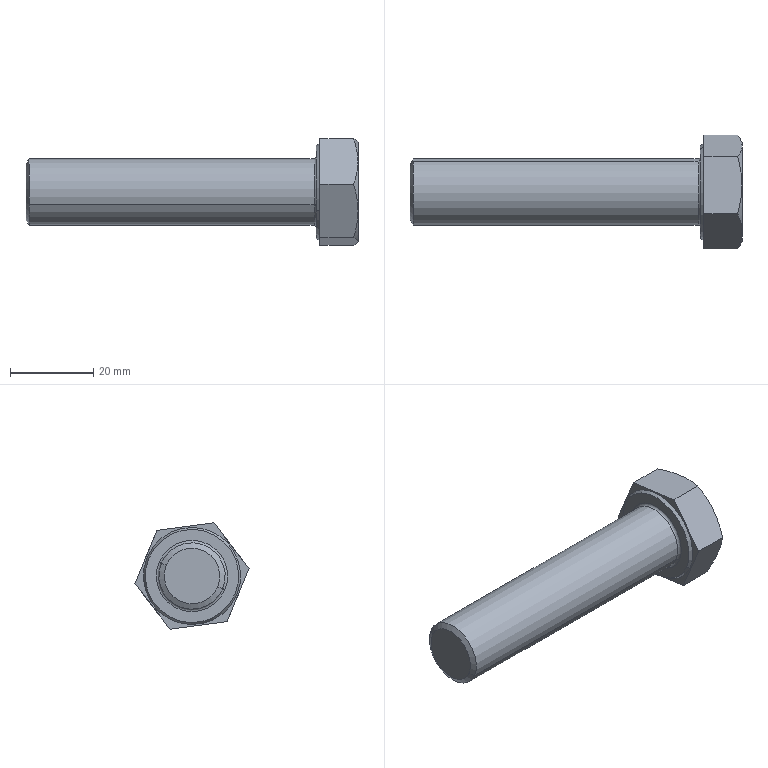Component | SolidWorks | GB_T5786-2000[HexHeadBoltFineThreadFullThreadM16_1.5_70]-1 | 1 solid | 24 faces | box 80 x 27.47 x 25.61 mm | volume 18960 mm3 | cone 10 | plane 10 | torus 2 | cylinder 2 | commonest cylinder face diameters 16 x2
STEP:
#1=COLOUR_RGB('',0.7922,0.8196,0.9333);
#2=FILL_AREA_STYLE_COLOUR('',#1);
#3=FILL_AREA_STYLE('',(#2));
#4=SURFACE_STYLE_FILL_AREA(#3);
#5=SURFACE_SIDE_STYLE('',(#4));
#6=SURFACE_STYLE_USAGE(.BOTH.,#5);
#7=PRESENTATION_STYLE_ASSIGNMENT((#6));
#8=CARTESIAN_POINT('',(-10.098,279.523,4.075));
#9=VERTEX_POINT('',#8);
#10=CARTESIAN_POINT('',(-10.098,280.01,4.277));
#11=VERTEX_POINT('',#10);
#12=CARTESIAN_POINT('',(-10.098,279.766,4.176));
#13=DIRECTION('',(1.,0.,0.));
#14=DIRECTION('',(0.,-0.9242,-0.3818));
#15=AXIS2_PLACEMENT_3D('',#12,#13,#14);
#16=CIRCLE('',#15,0.2638);
#17=EDGE_CURVE('',#9,#11,#16,.T.);
#18=ORIENTED_EDGE('',*,*,#17,.T.);
#19=CARTESIAN_POINT('',(-10.069,280.057,4.296));
#20=VERTEX_POINT('',#19);
#21=CARTESIAN_POINT('',(-10.069,280.057,4.296));
#22=DIRECTION('',(0.5,0.8004,0.3307));
#23=VECTOR('',#22,39.37);
#24=LINE('',#21,#23);
#25=EDGE_CURVE('',#11,#20,#24,.T.);
#26=ORIENTED_EDGE('',*,*,#25,.T.);
#27=CARTESIAN_POINT('',(-10.069,279.475,4.056));
#28=VERTEX_POINT('',#27);
#29=CARTESIAN_POINT('',(-10.069,279.766,4.176));
#30=DIRECTION('',(1.,0.,0.));
#31=DIRECTION('',(0.,-0.9242,-0.3818));
#32=AXIS2_PLACEMENT_3D('',#29,#30,#31);
#33=CIRCLE('',#32,0.315);
#34=EDGE_CURVE('',#28,#20,#33,.T.);
#35=ORIENTED_EDGE('',*,*,#34,.F.);
#36=CARTESIAN_POINT('',(-10.069,279.475,4.056));
#37=DIRECTION('',(0.5,-0.8004,-0.3307));
#38=VECTOR('',#37,39.37);
#39=LINE('',#36,#38);
#40=EDGE_CURVE('',#9,#28,#39,.T.);
#41=ORIENTED_EDGE('',*,*,#40,.F.);
#42=EDGE_LOOP('',(#18,#26,#35,#41));
#43=FACE_OUTER_BOUND('',#42,.T.);
#44=CARTESIAN_POINT('',(-10.069,279.766,4.176));
#45=DIRECTION('',(1.,0.,0.));
#46=DIRECTION('',(0.,-0.9242,-0.3818));
#47=AXIS2_PLACEMENT_3D('',#44,#45,#46);
#48=CONICAL_SURFACE('',#47,0.315,1.047);
#49=ADVANCED_FACE('',(#43),#48,.T.);
#50=CARTESIAN_POINT('',(-7.366,279.475,4.056));
#51=VERTEX_POINT('',#50);
#52=CARTESIAN_POINT('',(-7.366,280.057,4.296));
#53=VERTEX_POINT('',#52);
#54=CARTESIAN_POINT('',(-7.366,279.766,4.176));
#55=DIRECTION('',(-1.,0.,0.));
#56=DIRECTION('',(0.,0.9242,0.3818));
#57=AXIS2_PLACEMENT_3D('',#54,#55,#56);
#58=CIRCLE('',#57,0.315);
#59=EDGE_CURVE('',#51,#53,#58,.T.);
#60=ORIENTED_EDGE('',*,*,#59,.F.);
#61=CARTESIAN_POINT('',(-7.343,279.453,4.047));
#62=VERTEX_POINT('',#61);
#63=CARTESIAN_POINT('',(-7.366,279.453,4.047));
#64=DIRECTION('',(0.,0.3818,-0.9242));
#65=DIRECTION('',(0.,0.9242,0.3818));
#66=AXIS2_PLACEMENT_3D('',#63,#64,#65);
#67=CIRCLE('',#66,0.02362);
#68=EDGE_CURVE('',#51,#62,#67,.T.);
#69=ORIENTED_EDGE('',*,*,#68,.T.);
#70=CARTESIAN_POINT('',(-7.343,280.079,4.305));
#71=VERTEX_POINT('',#70);
#72=CARTESIAN_POINT('',(-7.343,279.766,4.176));
#73=DIRECTION('',(1.,0.,0.));
#74=DIRECTION('',(0.,0.9242,0.3818));
#75=AXIS2_PLACEMENT_3D('',#72,#73,#74);
#76=CIRCLE('',#75,0.3386);
#77=EDGE_CURVE('',#71,#62,#76,.T.);
#78=ORIENTED_EDGE('',*,*,#77,.F.);
#79=CARTESIAN_POINT('',(-7.366,280.079,4.305));
#80=DIRECTION('',(0.,-0.3818,0.9242));
#81=DIRECTION('',(0.,-0.9242,-0.3818));
#82=AXIS2_PLACEMENT_3D('',#79,#80,#81);
#83=CIRCLE('',#82,0.02362);
#84=EDGE_CURVE('',#53,#71,#83,.T.);
#85=ORIENTED_EDGE('',*,*,#84,.F.);
#86=EDGE_LOOP('',(#60,#69,#78,#85));
#87=FACE_OUTER_BOUND('',#86,.T.);
#88=CARTESIAN_POINT('',(-7.366,279.766,4.176));
#89=DIRECTION('',(-1.,0.,0.));
#90=DIRECTION('',(0.,0.9242,0.3818));
#91=AXIS2_PLACEMENT_3D('',#88,#89,#90);
#92=TOROIDAL_SURFACE('',#91,0.3386,0.02362);
#93=ADVANCED_FACE('',(#87),#92,.F.);
#94=CARTESIAN_POINT('',(-7.343,279.357,4.007));
#95=VERTEX_POINT('',#94);
#96=CARTESIAN_POINT('',(-7.343,280.176,4.345));
#97=VERTEX_POINT('',#96);
#98=CARTESIAN_POINT('',(-7.343,279.766,4.176));
#99=DIRECTION('',(1.,0.,0.));
#100=DIRECTION('',(0.,-0.9242,-0.3818));
#101=AXIS2_PLACEMENT_3D('',#98,#99,#100);
#102=CIRCLE('',#101,0.4427);
#103=EDGE_CURVE('',#95,#97,#102,.T.);
#104=ORIENTED_EDGE('',*,*,#103,.T.);
#105=CARTESIAN_POINT('',(-7.311,280.192,4.352));
#106=VERTEX_POINT('',#105);
#107=CARTESIAN_POINT('',(-7.311,280.192,4.352));
#108=DIRECTION('',(0.866,0.4621,0.1909));
#109=VECTOR('',#108,39.37);
#110=LINE('',#107,#109);
#111=EDGE_CURVE('',#97,#106,#110,.T.);
#112=ORIENTED_EDGE('',*,*,#111,.T.);
#113=CARTESIAN_POINT('',(-7.311,279.34,4.));
#114=VERTEX_POINT('',#113);
#115=CARTESIAN_POINT('',(-7.311,279.766,4.176));
#116=DIRECTION('',(1.,0.,0.));
#117=DIRECTION('',(0.,-0.9242,-0.3818));
#118=AXIS2_PLACEMENT_3D('',#115,#116,#117);
#119=CIRCLE('',#118,0.4609);
#120=EDGE_CURVE('',#114,#106,#119,.T.);
#121=ORIENTED_EDGE('',*,*,#120,.F.);
#122=CARTESIAN_POINT('',(-7.311,279.34,4.));
#123=DIRECTION('',(0.866,-0.4621,-0.1909));
#124=VECTOR('',#123,39.37);
#125=LINE('',#122,#124);
#126=EDGE_CURVE('',#95,#114,#125,.T.);
#127=ORIENTED_EDGE('',*,*,#126,.F.);
#128=EDGE_LOOP('',(#104,#112,#121,#127));
#129=FACE_OUTER_BOUND('',#128,.T.);
#130=CARTESIAN_POINT('',(-7.311,279.766,4.176));
#131=DIRECTION('',(1.,0.,0.));
#132=DIRECTION('',(0.,-0.9242,-0.3818));
#133=AXIS2_PLACEMENT_3D('',#130,#131,#132);
#134=CONICAL_SURFACE('',#133,0.4609,0.5236);
#135=ADVANCED_FACE('',(#129),#134,.T.);
#136=ORIENTED_EDGE('',*,*,#34,.T.);
#137=CARTESIAN_POINT('',(-6.949,280.057,4.296));
#138=DIRECTION('',(1.,0.,0.));
#139=VECTOR('',#138,39.37);
#140=LINE('',#137,#139);
#141=EDGE_CURVE('',#20,#53,#140,.T.);
#142=ORIENTED_EDGE('',*,*,#141,.T.);
#143=CARTESIAN_POINT('',(-7.366,279.766,4.176));
#144=DIRECTION('',(-1.,0.,0.));
#145=DIRECTION('',(0.,0.9242,0.3818));
#146=AXIS2_PLACEMENT_3D('',#143,#144,#145);
#147=CIRCLE('',#146,0.315);
#148=EDGE_CURVE('',#53,#51,#147,.T.);
#149=ORIENTED_EDGE('',*,*,#148,.T.);
#150=CARTESIAN_POINT('',(-6.949,279.475,4.056));
#151=DIRECTION('',(1.,0.,0.));
#152=VECTOR('',#151,39.37);
#153=LINE('',#150,#152);
#154=EDGE_CURVE('',#28,#51,#153,.T.);
#155=ORIENTED_EDGE('',*,*,#154,.F.);
#156=EDGE_LOOP('',(#136,#142,#149,#155));
#157=FACE_OUTER_BOUND('',#156,.T.);
#158=CARTESIAN_POINT('',(-6.949,279.766,4.176));
#159=DIRECTION('',(1.,0.,0.));
#160=DIRECTION('',(0.,-0.9242,-0.3818));
#161=AXIS2_PLACEMENT_3D('',#158,#159,#160);
#162=CYLINDRICAL_SURFACE('',#161,0.315);
#163=ADVANCED_FACE('',(#157),#162,.T.);
#164=ORIENTED_EDGE('',*,*,#141,.F.);
#165=CARTESIAN_POINT('',(-10.069,279.766,4.176));
#166=DIRECTION('',(1.,0.,0.));
#167=DIRECTION('',(0.,-0.9242,-0.3818));
#168=AXIS2_PLACEMENT_3D('',#165,#166,#167);
#169=CIRCLE('',#168,0.315);
#170=EDGE_CURVE('',#20,#28,#169,.T.);
#171=ORIENTED_EDGE('',*,*,#170,.T.);
#172=ORIENTED_EDGE('',*,*,#154,.T.);
#173=ORIENTED_EDGE('',*,*,#59,.T.);
#174=EDGE_LOOP('',(#164,#171,#172,#173));
#175=FACE_OUTER_BOUND('',#174,.T.);
#176=CARTESIAN_POINT('',(-6.949,279.766,4.176));
#177=DIRECTION('',(1.,0.,0.));
#178=DIRECTION('',(0.,-0.9242,-0.3818));
#179=AXIS2_PLACEMENT_3D('',#176,#177,#178);
#180=CYLINDRICAL_SURFACE('',#179,0.315);
#181=ADVANCED_FACE('',(#175),#180,.T.);
#182=CARTESIAN_POINT('',(-7.311,280.307,4.104));
#183=VERTEX_POINT('',#182);
#184=CARTESIAN_POINT('',(-7.311,279.975,3.672));
#185=VERTEX_POINT('',#184);
#186=CARTESIAN_POINT('',(-7.311,280.307,4.104));
#187=DIRECTION('',(0.,-0.6095,-0.7928));
#188=VECTOR('',#187,39.37);
#189=LINE('',#186,#188);
#190=EDGE_CURVE('',#183,#185,#189,.T.);
#191=ORIENTED_EDGE('',*,*,#190,.F.);
#192=CARTESIAN_POINT('',(-6.991,280.307,4.104));
#193=VERTEX_POINT('',#192);
#194=CARTESIAN_POINT('',(-7.343,280.307,4.104));
#195=DIRECTION('',(1.,0.,0.));
#196=VECTOR('',#195,39.37);
#197=LINE('',#194,#196);
#198=EDGE_CURVE('',#183,#193,#197,.T.);
#199=ORIENTED_EDGE('',*,*,#198,.T.);
#200=CARTESIAN_POINT('',(-6.949,280.141,3.888));
#201=VERTEX_POINT('',#200);
#202=CARTESIAN_POINT('',(-6.949,280.141,3.888));
#203=CARTESIAN_POINT('',(-6.949,280.155,3.906));
#204=CARTESIAN_POINT('',(-6.95,280.169,3.925));
#205=CARTESIAN_POINT('',(-6.954,280.197,3.961));
#206=CARTESIAN_POINT('',(-6.957,280.211,3.979));
#207=CARTESIAN_POINT('',(-6.968,280.253,4.033));
#208=CARTESIAN_POINT('',(-6.978,280.28,4.069));
#209=CARTESIAN_POINT('',(-6.991,280.307,4.104));
#210=B_SPLINE_CURVE_WITH_KNOTS('',3,(#202,#203,#204,#205,#206,#207,#208,#209),.UNSPECIFIED.,.F.,.F.,(4,2,2,4),(0.00701,0.008756,0.0105,0.01399),.UNSPECIFIED.);
#211=EDGE_CURVE('',#201,#193,#210,.T.);
#212=ORIENTED_EDGE('',*,*,#211,.F.);
#213=CARTESIAN_POINT('',(-6.991,279.975,3.672));
#214=VERTEX_POINT('',#213);
#215=CARTESIAN_POINT('',(-6.991,279.975,3.672));
#216=CARTESIAN_POINT('',(-6.978,280.002,3.707));
#217=CARTESIAN_POINT('',(-6.968,280.029,3.743));
#218=CARTESIAN_POINT('',(-6.953,280.085,3.815));
#219=CARTESIAN_POINT('',(-6.949,280.113,3.851));
#220=CARTESIAN_POINT('',(-6.949,280.141,3.888));
#221=B_SPLINE_CURVE_WITH_KNOTS('',3,(#215,#216,#217,#218,#219,#220),.UNSPECIFIED.,.F.,.F.,(4,2,4),(0.00000024,0.003505,0.00701),.UNSPECIFIED.);
#222=EDGE_CURVE('',#214,#201,#221,.T.);
#223=ORIENTED_EDGE('',*,*,#222,.F.);
#224=CARTESIAN_POINT('',(-7.343,279.975,3.672));
#225=DIRECTION('',(1.,0.,0.));
#226=VECTOR('',#225,39.37);
#227=LINE('',#224,#226);
#228=EDGE_CURVE('',#185,#214,#227,.T.);
#229=ORIENTED_EDGE('',*,*,#228,.F.);
#230=EDGE_LOOP('',(#191,#199,#212,#223,#229));
#231=FACE_OUTER_BOUND('',#230,.T.);
#232=CARTESIAN_POINT('',(-7.343,280.307,4.104));
#233=DIRECTION('',(0.,-0.7928,0.6095));
#234=DIRECTION('',(0.,0.6095,0.7928));
#235=AXIS2_PLACEMENT_3D('',#232,#233,#234);
#236=PLANE('',#235);
#237=ADVANCED_FACE('',(#231),#236,.F.);
#238=CARTESIAN_POINT('',(-7.311,279.434,3.743));
#239=VERTEX_POINT('',#238);
#240=CARTESIAN_POINT('',(-7.311,279.975,3.672));
#241=DIRECTION('',(0.,-0.9913,0.1314));
#242=VECTOR('',#241,39.37);
#243=LINE('',#240,#242);
#244=EDGE_CURVE('',#185,#239,#243,.T.);
#245=ORIENTED_EDGE('',*,*,#244,.F.);
#246=ORIENTED_EDGE('',*,*,#228,.T.);
#247=CARTESIAN_POINT('',(-6.949,279.704,3.707));
#248=VERTEX_POINT('',#247);
#249=CARTESIAN_POINT('',(-6.949,279.704,3.707));
#250=CARTESIAN_POINT('',(-6.949,279.727,3.704));
#251=CARTESIAN_POINT('',(-6.95,279.75,3.701));
#252=CARTESIAN_POINT('',(-6.954,279.796,3.695));
#253=CARTESIAN_POINT('',(-6.957,279.819,3.692));
#254=CARTESIAN_POINT('',(-6.968,279.886,3.683));
#255=CARTESIAN_POINT('',(-6.978,279.931,3.677));
#256=CARTESIAN_POINT('',(-6.991,279.975,3.672));
#257=B_SPLINE_CURVE_WITH_KNOTS('',3,(#249,#250,#251,#252,#253,#254,#255,#256),.UNSPECIFIED.,.F.,.F.,(4,2,2,4),(0.00701,0.008756,0.0105,0.01399),.UNSPECIFIED.);
#258=EDGE_CURVE('',#248,#214,#257,.T.);
#259=ORIENTED_EDGE('',*,*,#258,.F.);
#260=CARTESIAN_POINT('',(-6.991,279.434,3.743));
#261=VERTEX_POINT('',#260);
#262=CARTESIAN_POINT('',(-6.991,279.434,3.743));
#263=CARTESIAN_POINT('',(-6.978,279.478,3.737));
#264=CARTESIAN_POINT('',(-6.968,279.523,3.732));
#265=CARTESIAN_POINT('',(-6.953,279.613,3.72));
#266=CARTESIAN_POINT('',(-6.949,279.658,3.714));
#267=CARTESIAN_POINT('',(-6.949,279.704,3.707));
#268=B_SPLINE_CURVE_WITH_KNOTS('',3,(#262,#263,#264,#265,#266,#267),.UNSPECIFIED.,.F.,.F.,(4,2,4),(0.00000024,0.003505,0.00701),.UNSPECIFIED.);
#269=EDGE_CURVE('',#261,#248,#268,.T.);
#270=ORIENTED_EDGE('',*,*,#269,.F.);
#271=CARTESIAN_POINT('',(-7.343,279.434,3.743));
#272=DIRECTION('',(1.,0.,0.));
#273=VECTOR('',#272,39.37);
#274=LINE('',#271,#273);
#275=EDGE_CURVE('',#239,#261,#274,.T.);
#276=ORIENTED_EDGE('',*,*,#275,.F.);
#277=EDGE_LOOP('',(#245,#246,#259,#270,#276));
#278=FACE_OUTER_BOUND('',#277,.T.);
#279=CARTESIAN_POINT('',(-7.343,279.975,3.672));
#280=DIRECTION('',(0.,0.1314,0.9913));
#281=DIRECTION('',(0.,0.9913,-0.1314));
#282=AXIS2_PLACEMENT_3D('',#279,#280,#281);
#283=PLANE('',#282);
#284=ADVANCED_FACE('',(#278),#283,.F.);
#285=CARTESIAN_POINT('',(-7.311,279.226,4.248));
#286=VERTEX_POINT('',#285);
#287=CARTESIAN_POINT('',(-7.311,279.434,3.743));
#288=DIRECTION('',(0.,-0.3818,0.9242));
#289=VECTOR('',#288,39.37);
#290=LINE('',#287,#289);
#291=EDGE_CURVE('',#239,#286,#290,.T.);
#292=ORIENTED_EDGE('',*,*,#291,.F.);
#293=ORIENTED_EDGE('',*,*,#275,.T.);
#294=CARTESIAN_POINT('',(-6.949,279.33,3.995));
#295=VERTEX_POINT('',#294);
#296=CARTESIAN_POINT('',(-6.949,279.33,3.995));
#297=CARTESIAN_POINT('',(-6.949,279.339,3.974));
#298=CARTESIAN_POINT('',(-6.95,279.347,3.953));
#299=CARTESIAN_POINT('',(-6.954,279.365,3.91));
#300=CARTESIAN_POINT('',(-6.957,279.374,3.888));
#301=CARTESIAN_POINT('',(-6.968,279.4,3.825));
#302=CARTESIAN_POINT('',(-6.978,279.417,3.784));
#303=CARTESIAN_POINT('',(-6.991,279.434,3.743));
#304=B_SPLINE_CURVE_WITH_KNOTS('',3,(#296,#297,#298,#299,#300,#301,#302,#303),.UNSPECIFIED.,.F.,.F.,(4,2,2,4),(0.01982,0.02158,0.02333,0.02684),.UNSPECIFIED.);
#305=EDGE_CURVE('',#295,#261,#304,.T.);
#306=ORIENTED_EDGE('',*,*,#305,.F.);
#307=CARTESIAN_POINT('',(-6.991,279.226,4.248));
#308=VERTEX_POINT('',#307);
#309=CARTESIAN_POINT('',(-6.991,279.226,4.248));
#310=CARTESIAN_POINT('',(-6.978,279.243,4.206));
#311=CARTESIAN_POINT('',(-6.967,279.26,4.165));
#312=CARTESIAN_POINT('',(-6.953,279.295,4.08));
#313=CARTESIAN_POINT('',(-6.949,279.312,4.038));
#314=CARTESIAN_POINT('',(-6.949,279.33,3.995));
#315=B_SPLINE_CURVE_WITH_KNOTS('',3,(#309,#310,#311,#312,#313,#314),.UNSPECIFIED.,.F.,.F.,(4,2,4),(0.01281,0.01632,0.01982),.UNSPECIFIED.);
#316=EDGE_CURVE('',#308,#295,#315,.T.);
#317=ORIENTED_EDGE('',*,*,#316,.F.);
#318=CARTESIAN_POINT('',(-7.343,279.226,4.248));
#319=DIRECTION('',(1.,0.,0.));
#320=VECTOR('',#319,39.37);
#321=LINE('',#318,#320);
#322=EDGE_CURVE('',#286,#308,#321,.T.);
#323=ORIENTED_EDGE('',*,*,#322,.F.);
#324=EDGE_LOOP('',(#292,#293,#306,#317,#323));
#325=FACE_OUTER_BOUND('',#324,.T.);
#326=CARTESIAN_POINT('',(-7.343,279.434,3.743));
#327=DIRECTION('',(0.,0.9242,0.3818));
#328=DIRECTION('',(1.,0.,0.));
#329=AXIS2_PLACEMENT_3D('',#326,#327,#328);
#330=PLANE('',#329);
#331=ADVANCED_FACE('',(#325),#330,.F.);
#332=CARTESIAN_POINT('',(-7.311,279.558,4.68));
#333=VERTEX_POINT('',#332);
#334=CARTESIAN_POINT('',(-7.311,279.558,4.68));
#335=DIRECTION('',(0.,0.6095,0.7928));
#336=VECTOR('',#335,39.37);
#337=LINE('',#334,#336);
#338=EDGE_CURVE('',#286,#333,#337,.T.);
#339=ORIENTED_EDGE('',*,*,#338,.F.);
#340=ORIENTED_EDGE('',*,*,#322,.T.);
#341=CARTESIAN_POINT('',(-6.949,279.392,4.464));
#342=VERTEX_POINT('',#341);
#343=CARTESIAN_POINT('',(-6.949,279.392,4.464));
#344=CARTESIAN_POINT('',(-6.949,279.378,4.445));
#345=CARTESIAN_POINT('',(-6.95,279.364,4.427));
#346=CARTESIAN_POINT('',(-6.954,279.336,4.391));
#347=CARTESIAN_POINT('',(-6.957,279.322,4.372));
#348=CARTESIAN_POINT('',(-6.968,279.28,4.318));
#349=CARTESIAN_POINT('',(-6.978,279.253,4.283));
#350=CARTESIAN_POINT('',(-6.991,279.226,4.248));
#351=B_SPLINE_CURVE_WITH_KNOTS('',3,(#343,#344,#345,#346,#347,#348,#349,#350),.UNSPECIFIED.,.F.,.F.,(4,2,2,4),(0.00701,0.008756,0.0105,0.01399),.UNSPECIFIED.);
#352=EDGE_CURVE('',#342,#308,#351,.T.);
#353=ORIENTED_EDGE('',*,*,#352,.F.);
#354=CARTESIAN_POINT('',(-6.991,279.558,4.68));
#355=VERTEX_POINT('',#354);
#356=CARTESIAN_POINT('',(-6.991,279.558,4.68));
#357=CARTESIAN_POINT('',(-6.978,279.531,4.645));
#358=CARTESIAN_POINT('',(-6.968,279.503,4.609));
#359=CARTESIAN_POINT('',(-6.953,279.448,4.537));
#360=CARTESIAN_POINT('',(-6.949,279.42,4.501));
#361=CARTESIAN_POINT('',(-6.949,279.392,4.464));
#362=B_SPLINE_CURVE_WITH_KNOTS('',3,(#356,#357,#358,#359,#360,#361),.UNSPECIFIED.,.F.,.F.,(4,2,4),(0.00000024,0.003505,0.00701),.UNSPECIFIED.);
#363=EDGE_CURVE('',#355,#342,#362,.T.);
#364=ORIENTED_EDGE('',*,*,#363,.F.);
#365=CARTESIAN_POINT('',(-7.343,279.558,4.68));
#366=DIRECTION('',(1.,0.,0.));
#367=VECTOR('',#366,39.37);
#368=LINE('',#365,#367);
#369=EDGE_CURVE('',#333,#355,#368,.T.);
#370=ORIENTED_EDGE('',*,*,#369,.F.);
#371=EDGE_LOOP('',(#339,#340,#353,#364,#370));
#372=FACE_OUTER_BOUND('',#371,.T.);
#373=CARTESIAN_POINT('',(-7.343,279.558,4.68));
#374=DIRECTION('',(0.,0.7928,-0.6095));
#375=DIRECTION('',(0.,-0.6095,-0.7928));
#376=AXIS2_PLACEMENT_3D('',#373,#374,#375);
#377=PLANE('',#376);
#378=ADVANCED_FACE('',(#372),#377,.F.);
#379=CARTESIAN_POINT('',(-7.311,280.099,4.608));
#380=VERTEX_POINT('',#379);
#381=CARTESIAN_POINT('',(-7.311,280.099,4.608));
#382=DIRECTION('',(0.,0.9913,-0.1314));
#383=VECTOR('',#382,39.37);
#384=LINE('',#381,#383);
#385=EDGE_CURVE('',#333,#380,#384,.T.);
#386=ORIENTED_EDGE('',*,*,#385,.F.);
#387=ORIENTED_EDGE('',*,*,#369,.T.);
#388=CARTESIAN_POINT('',(-6.949,279.828,4.644));
#389=VERTEX_POINT('',#388);
#390=CARTESIAN_POINT('',(-6.949,279.828,4.644));
#391=CARTESIAN_POINT('',(-6.949,279.806,4.647));
#392=CARTESIAN_POINT('',(-6.95,279.782,4.65));
#393=CARTESIAN_POINT('',(-6.954,279.737,4.656));
#394=CARTESIAN_POINT('',(-6.957,279.714,4.659));
#395=CARTESIAN_POINT('',(-6.968,279.647,4.668));
#396=CARTESIAN_POINT('',(-6.978,279.602,4.674));
#397=CARTESIAN_POINT('',(-6.991,279.558,4.68));
#398=B_SPLINE_CURVE_WITH_KNOTS('',3,(#390,#391,#392,#393,#394,#395,#396,#397),.UNSPECIFIED.,.F.,.F.,(4,2,2,4),(0.00701,0.008756,0.0105,0.01399),.UNSPECIFIED.);
#399=EDGE_CURVE('',#389,#355,#398,.T.);
#400=ORIENTED_EDGE('',*,*,#399,.F.);
#401=CARTESIAN_POINT('',(-6.991,280.099,4.608));
#402=VERTEX_POINT('',#401);
#403=CARTESIAN_POINT('',(-6.991,280.099,4.608));
#404=CARTESIAN_POINT('',(-6.978,280.055,4.614));
#405=CARTESIAN_POINT('',(-6.968,280.01,4.62));
#406=CARTESIAN_POINT('',(-6.953,279.92,4.632));
#407=CARTESIAN_POINT('',(-6.949,279.875,4.638));
#408=CARTESIAN_POINT('',(-6.949,279.828,4.644));
#409=B_SPLINE_CURVE_WITH_KNOTS('',3,(#403,#404,#405,#406,#407,#408),.UNSPECIFIED.,.F.,.F.,(4,2,4),(0.00000024,0.003505,0.00701),.UNSPECIFIED.);
#410=EDGE_CURVE('',#402,#389,#409,.T.);
#411=ORIENTED_EDGE('',*,*,#410,.F.);
#412=CARTESIAN_POINT('',(-7.343,280.099,4.608));
#413=DIRECTION('',(1.,0.,0.));
#414=VECTOR('',#413,39.37);
#415=LINE('',#412,#414);
#416=EDGE_CURVE('',#380,#402,#415,.T.);
#417=ORIENTED_EDGE('',*,*,#416,.F.);
#418=EDGE_LOOP('',(#386,#387,#400,#411,#417));
#419=FACE_OUTER_BOUND('',#418,.T.);
#420=CARTESIAN_POINT('',(-7.343,280.099,4.608));
#421=DIRECTION('',(0.,-0.1314,-0.9913));
#422=DIRECTION('',(0.,-0.9913,0.1314));
#423=AXIS2_PLACEMENT_3D('',#420,#421,#422);
#424=PLANE('',#423);
#425=ADVANCED_FACE('',(#419),#424,.F.);
#426=CARTESIAN_POINT('',(-7.311,280.307,4.104));
#427=DIRECTION('',(0.,0.3818,-0.9242));
#428=VECTOR('',#427,39.37);
#429=LINE('',#426,#428);
#430=EDGE_CURVE('',#380,#183,#429,.T.);
#431=ORIENTED_EDGE('',*,*,#430,.F.);
#432=ORIENTED_EDGE('',*,*,#416,.T.);
#433=CARTESIAN_POINT('',(-6.949,280.203,4.356));
#434=VERTEX_POINT('',#433);
#435=CARTESIAN_POINT('',(-6.949,280.203,4.356));
#436=CARTESIAN_POINT('',(-6.949,280.185,4.399));
#437=CARTESIAN_POINT('',(-6.953,280.168,4.441));
#438=CARTESIAN_POINT('',(-6.967,280.133,4.525));
#439=CARTESIAN_POINT('',(-6.978,280.116,4.567));
#440=CARTESIAN_POINT('',(-6.991,280.099,4.608));
#441=B_SPLINE_CURVE_WITH_KNOTS('',3,(#435,#436,#437,#438,#439,#440),.UNSPECIFIED.,.F.,.F.,(4,2,4),(0.03938,0.04289,0.0464),.UNSPECIFIED.);
#442=EDGE_CURVE('',#434,#402,#441,.T.);
#443=ORIENTED_EDGE('',*,*,#442,.F.);
#444=CARTESIAN_POINT('',(-6.991,280.307,4.104));
#445=CARTESIAN_POINT('',(-6.978,280.29,4.145));
#446=CARTESIAN_POINT('',(-6.968,280.273,4.186));
#447=CARTESIAN_POINT('',(-6.957,280.247,4.249));
#448=CARTESIAN_POINT('',(-6.954,280.238,4.271));
#449=CARTESIAN_POINT('',(-6.95,280.221,4.313));
#450=CARTESIAN_POINT('',(-6.949,280.212,4.335));
#451=CARTESIAN_POINT('',(-6.949,280.203,4.356));
#452=B_SPLINE_CURVE_WITH_KNOTS('',3,(#444,#445,#446,#447,#448,#449,#450,#451),.UNSPECIFIED.,.F.,.F.,(4,2,2,4),(0.03236,0.03587,0.03763,0.03938),.UNSPECIFIED.);
#453=EDGE_CURVE('',#193,#434,#452,.T.);
#454=ORIENTED_EDGE('',*,*,#453,.F.);
#455=ORIENTED_EDGE('',*,*,#198,.F.);
#456=EDGE_LOOP('',(#431,#432,#443,#454,#455));
#457=FACE_OUTER_BOUND('',#456,.T.);
#458=CARTESIAN_POINT('',(-7.343,280.307,4.104));
#459=DIRECTION('',(0.,-0.9242,-0.3818));
#460=DIRECTION('',(-1.,0.,0.));
#461=AXIS2_PLACEMENT_3D('',#458,#459,#460);
#462=PLANE('',#461);
#463=ADVANCED_FACE('',(#457),#462,.F.);
#464=ORIENTED_EDGE('',*,*,#410,.T.);
#465=CARTESIAN_POINT('',(-6.949,279.766,4.176));
#466=DIRECTION('',(-1.,0.,0.));
#467=DIRECTION('',(0.,0.9242,0.3818));
#468=AXIS2_PLACEMENT_3D('',#465,#466,#467);
#469=CIRCLE('',#468,0.4724);
#470=EDGE_CURVE('',#389,#434,#469,.T.);
#471=ORIENTED_EDGE('',*,*,#470,.T.);
#472=ORIENTED_EDGE('',*,*,#442,.T.);
#473=EDGE_LOOP('',(#464,#471,#472));
#474=FACE_OUTER_BOUND('',#473,.T.);
#475=CARTESIAN_POINT('',(-6.949,279.766,4.176));
#476=DIRECTION('',(-1.,0.,0.));
#477=DIRECTION('',(0.,0.9242,0.3818));
#478=AXIS2_PLACEMENT_3D('',#475,#476,#477);
#479=CONICAL_SURFACE('',#478,0.4724,1.047);
#480=ADVANCED_FACE('',(#474),#479,.T.);
#481=ORIENTED_EDGE('',*,*,#363,.T.);
#482=CARTESIAN_POINT('',(-6.949,279.766,4.176));
#483=DIRECTION('',(-1.,0.,0.));
#484=DIRECTION('',(0.,0.9242,0.3818));
#485=AXIS2_PLACEMENT_3D('',#482,#483,#484);
#486=CIRCLE('',#485,0.4724);
#487=EDGE_CURVE('',#342,#389,#486,.T.);
#488=ORIENTED_EDGE('',*,*,#487,.T.);
#489=ORIENTED_EDGE('',*,*,#399,.T.);
#490=EDGE_LOOP('',(#481,#488,#489));
#491=FACE_OUTER_BOUND('',#490,.T.);
#492=CARTESIAN_POINT('',(-6.949,279.766,4.176));
#493=DIRECTION('',(-1.,0.,0.));
#494=DIRECTION('',(0.,0.9242,0.3818));
#495=AXIS2_PLACEMENT_3D('',#492,#493,#494);
#496=CONICAL_SURFACE('',#495,0.4724,1.047);
#497=ADVANCED_FACE('',(#491),#496,.T.);
#498=ORIENTED_EDGE('',*,*,#316,.T.);
#499=CARTESIAN_POINT('',(-6.949,279.766,4.176));
#500=DIRECTION('',(-1.,0.,0.));
#501=DIRECTION('',(0.,0.9242,0.3818));
#502=AXIS2_PLACEMENT_3D('',#499,#500,#501);
#503=CIRCLE('',#502,0.4724);
#504=EDGE_CURVE('',#295,#342,#503,.T.);
#505=ORIENTED_EDGE('',*,*,#504,.T.);
#506=ORIENTED_EDGE('',*,*,#352,.T.);
#507=EDGE_LOOP('',(#498,#505,#506));
#508=FACE_OUTER_BOUND('',#507,.T.);
#509=CARTESIAN_POINT('',(-6.949,279.766,4.176));
#510=DIRECTION('',(-1.,0.,0.));
#511=DIRECTION('',(0.,0.9242,0.3818));
#512=AXIS2_PLACEMENT_3D('',#509,#510,#511);
#513=CONICAL_SURFACE('',#512,0.4724,1.047);
#514=ADVANCED_FACE('',(#508),#513,.T.);
#515=ORIENTED_EDGE('',*,*,#305,.T.);
#516=ORIENTED_EDGE('',*,*,#269,.T.);
#517=CARTESIAN_POINT('',(-6.949,279.766,4.176));
#518=DIRECTION('',(1.,0.,0.));
#519=DIRECTION('',(0.,-0.9242,-0.3818));
#520=AXIS2_PLACEMENT_3D('',#517,#518,#519);
#521=CIRCLE('',#520,0.4724);
#522=EDGE_CURVE('',#295,#248,#521,.T.);
#523=ORIENTED_EDGE('',*,*,#522,.F.);
#524=EDGE_LOOP('',(#515,#516,#523));
#525=FACE_OUTER_BOUND('',#524,.T.);
#526=CARTESIAN_POINT('',(-6.949,279.766,4.176));
#527=DIRECTION('',(-1.,0.,0.));
#528=DIRECTION('',(0.,0.9242,0.3818));
#529=AXIS2_PLACEMENT_3D('',#526,#527,#528);
#530=CONICAL_SURFACE('',#529,0.4724,1.047);
#531=ADVANCED_FACE('',(#525),#530,.T.);
#532=ORIENTED_EDGE('',*,*,#258,.T.);
#533=ORIENTED_EDGE('',*,*,#222,.T.);
#534=CARTESIAN_POINT('',(-6.949,279.766,4.176));
#535=DIRECTION('',(-1.,0.,0.));
#536=DIRECTION('',(0.,0.9242,0.3818));
#537=AXIS2_PLACEMENT_3D('',#534,#535,#536);
#538=CIRCLE('',#537,0.4724);
#539=EDGE_CURVE('',#201,#248,#538,.T.);
#540=ORIENTED_EDGE('',*,*,#539,.T.);
#541=EDGE_LOOP('',(#532,#533,#540));
#542=FACE_OUTER_BOUND('',#541,.T.);
#543=CARTESIAN_POINT('',(-6.949,279.766,4.176));
#544=DIRECTION('',(-1.,0.,0.));
#545=DIRECTION('',(0.,0.9242,0.3818));
#546=AXIS2_PLACEMENT_3D('',#543,#544,#545);
#547=CONICAL_SURFACE('',#546,0.4724,1.047);
#548=ADVANCED_FACE('',(#542),#547,.T.);
#549=ORIENTED_EDGE('',*,*,#211,.T.);
#550=ORIENTED_EDGE('',*,*,#453,.T.);
#551=CARTESIAN_POINT('',(-6.949,279.766,4.176));
#552=DIRECTION('',(-1.,0.,0.));
#553=DIRECTION('',(0.,0.9242,0.3818));
#554=AXIS2_PLACEMENT_3D('',#551,#552,#553);
#555=CIRCLE('',#554,0.4724);
#556=EDGE_CURVE('',#434,#201,#555,.T.);
#557=ORIENTED_EDGE('',*,*,#556,.T.);
#558=EDGE_LOOP('',(#549,#550,#557));
#559=FACE_OUTER_BOUND('',#558,.T.);
#560=CARTESIAN_POINT('',(-6.949,279.766,4.176));
#561=DIRECTION('',(-1.,0.,0.));
#562=DIRECTION('',(0.,0.9242,0.3818));
#563=AXIS2_PLACEMENT_3D('',#560,#561,#562);
#564=CONICAL_SURFACE('',#563,0.4724,1.047);
#565=ADVANCED_FACE('',(#559),#564,.T.);
#566=ORIENTED_EDGE('',*,*,#556,.F.);
#567=ORIENTED_EDGE('',*,*,#470,.F.);
#568=ORIENTED_EDGE('',*,*,#487,.F.);
#569=ORIENTED_EDGE('',*,*,#504,.F.);
#570=ORIENTED_EDGE('',*,*,#522,.T.);
#571=ORIENTED_EDGE('',*,*,#539,.F.);
#572=EDGE_LOOP('',(#566,#567,#568,#569,#570,#571));
#573=FACE_OUTER_BOUND('',#572,.T.);
#574=CARTESIAN_POINT('',(-6.949,280.64,4.537));
#575=DIRECTION('',(-1.,0.,0.));
#576=DIRECTION('',(0.,0.9242,0.3818));
#577=AXIS2_PLACEMENT_3D('',#574,#575,#576);
#578=PLANE('',#577);
#579=ADVANCED_FACE('',(#573),#578,.F.);
#580=ORIENTED_EDGE('',*,*,#120,.T.);
#581=CARTESIAN_POINT('',(-7.311,279.766,4.176));
#582=DIRECTION('',(1.,0.,0.));
#583=DIRECTION('',(0.,-0.9242,-0.3818));
#584=AXIS2_PLACEMENT_3D('',#581,#582,#583);
#585=CIRCLE('',#584,0.4609);
#586=EDGE_CURVE('',#106,#114,#585,.T.);
#587=ORIENTED_EDGE('',*,*,#586,.T.);
#588=EDGE_LOOP('',(#580,#587));
#589=FACE_BOUND('',#588,.T.);
#590=ORIENTED_EDGE('',*,*,#190,.T.);
#591=ORIENTED_EDGE('',*,*,#244,.T.);
#592=ORIENTED_EDGE('',*,*,#291,.T.);
#593=ORIENTED_EDGE('',*,*,#338,.T.);
#594=ORIENTED_EDGE('',*,*,#385,.T.);
#595=ORIENTED_EDGE('',*,*,#430,.T.);
#596=EDGE_LOOP('',(#590,#591,#592,#593,#594,#595));
#597=FACE_OUTER_BOUND('',#596,.T.);
#598=CARTESIAN_POINT('',(-7.311,279.942,3.75));
#599=DIRECTION('',(-1.,0.,0.));
#600=DIRECTION('',(0.,0.9242,0.3818));
#601=AXIS2_PLACEMENT_3D('',#598,#599,#600);
#602=PLANE('',#601);
#603=ADVANCED_FACE('',(#589,#597),#602,.T.);
#604=ORIENTED_EDGE('',*,*,#111,.F.);
#605=CARTESIAN_POINT('',(-7.343,279.766,4.176));
#606=DIRECTION('',(1.,0.,0.));
#607=DIRECTION('',(0.,-0.9242,-0.3818));
#608=AXIS2_PLACEMENT_3D('',#605,#606,#607);
#609=CIRCLE('',#608,0.4427);
#610=EDGE_CURVE('',#97,#95,#609,.T.);
#611=ORIENTED_EDGE('',*,*,#610,.T.);
#612=ORIENTED_EDGE('',*,*,#126,.T.);
#613=ORIENTED_EDGE('',*,*,#586,.F.);
#614=EDGE_LOOP('',(#604,#611,#612,#613));
#615=FACE_OUTER_BOUND('',#614,.T.);
#616=CARTESIAN_POINT('',(-7.311,279.766,4.176));
#617=DIRECTION('',(1.,0.,0.));
#618=DIRECTION('',(0.,-0.9242,-0.3818));
#619=AXIS2_PLACEMENT_3D('',#616,#617,#618);
#620=CONICAL_SURFACE('',#619,0.4609,0.5236);
#621=ADVANCED_FACE('',(#615),#620,.T.);
#622=ORIENTED_EDGE('',*,*,#77,.T.);
#623=CARTESIAN_POINT('',(-7.343,279.766,4.176));
#624=DIRECTION('',(1.,0.,0.));
#625=DIRECTION('',(0.,0.9242,0.3818));
#626=AXIS2_PLACEMENT_3D('',#623,#624,#625);
#627=CIRCLE('',#626,0.3386);
#628=EDGE_CURVE('',#62,#71,#627,.T.);
#629=ORIENTED_EDGE('',*,*,#628,.T.);
#630=EDGE_LOOP('',(#622,#629));
#631=FACE_BOUND('',#630,.T.);
#632=ORIENTED_EDGE('',*,*,#103,.F.);
#633=ORIENTED_EDGE('',*,*,#610,.F.);
#634=EDGE_LOOP('',(#632,#633));
#635=FACE_OUTER_BOUND('',#634,.T.);
#636=CARTESIAN_POINT('',(-7.343,280.64,4.537));
#637=DIRECTION('',(-1.,0.,0.));
#638=DIRECTION('',(0.,0.9242,0.3818));
#639=AXIS2_PLACEMENT_3D('',#636,#637,#638);
#640=PLANE('',#639);
#641=ADVANCED_FACE('',(#631,#635),#640,.T.);
#642=ORIENTED_EDGE('',*,*,#68,.F.);
#643=ORIENTED_EDGE('',*,*,#148,.F.);
#644=ORIENTED_EDGE('',*,*,#84,.T.);
#645=ORIENTED_EDGE('',*,*,#628,.F.);
#646=EDGE_LOOP('',(#642,#643,#644,#645));
#647=FACE_OUTER_BOUND('',#646,.T.);
#648=CARTESIAN_POINT('',(-7.366,279.766,4.176));
#649=DIRECTION('',(-1.,0.,0.));
#650=DIRECTION('',(0.,0.9242,0.3818));
#651=AXIS2_PLACEMENT_3D('',#648,#649,#650);
#652=TOROIDAL_SURFACE('',#651,0.3386,0.02362);
#653=ADVANCED_FACE('',(#647),#652,.F.);
#654=ORIENTED_EDGE('',*,*,#25,.F.);
#655=CARTESIAN_POINT('',(-10.098,279.766,4.176));
#656=DIRECTION('',(1.,0.,0.));
#657=DIRECTION('',(0.,-0.9242,-0.3818));
#658=AXIS2_PLACEMENT_3D('',#655,#656,#657);
#659=CIRCLE('',#658,0.2638);
#660=EDGE_CURVE('',#11,#9,#659,.T.);
#661=ORIENTED_EDGE('',*,*,#660,.T.);
#662=ORIENTED_EDGE('',*,*,#40,.T.);
#663=ORIENTED_EDGE('',*,*,#170,.F.);
#664=EDGE_LOOP('',(#654,#661,#662,#663));
#665=FACE_OUTER_BOUND('',#664,.T.);
#666=CARTESIAN_POINT('',(-10.069,279.766,4.176));
#667=DIRECTION('',(1.,0.,0.));
#668=DIRECTION('',(0.,-0.9242,-0.3818));
#669=AXIS2_PLACEMENT_3D('',#666,#667,#668);
#670=CONICAL_SURFACE('',#669,0.315,1.047);
#671=ADVANCED_FACE('',(#665),#670,.T.);
#672=ORIENTED_EDGE('',*,*,#17,.F.);
#673=ORIENTED_EDGE('',*,*,#660,.F.);
#674=EDGE_LOOP('',(#672,#673));
#675=FACE_OUTER_BOUND('',#674,.T.);
#676=CARTESIAN_POINT('',(-10.098,279.766,4.176));
#677=DIRECTION('',(1.,0.,0.));
#678=DIRECTION('',(0.,-0.9242,-0.3818));
#679=AXIS2_PLACEMENT_3D('',#676,#677,#678);
#680=PLANE('',#679);
#681=ADVANCED_FACE('',(#675),#680,.F.);
#682=CLOSED_SHELL('',(#49,#93,#135,#163,#181,#237,#284,#331,#378,#425,#463,#480,#497,#514,#531,#548,#565,#579,#603,#621,#641,#653,#671,#681));
#683=MANIFOLD_SOLID_BREP('',#682);
#684=STYLED_ITEM('',(#7),#683);
#685=(LENGTH_UNIT()NAMED_UNIT(*)SI_UNIT($,.METRE.));
#686=LENGTH_MEASURE_WITH_UNIT(LENGTH_MEASURE(0.0254),#685);
#687=DIMENSIONAL_EXPONENTS(1.,0.,0.,0.,0.,0.,0.);
#688=(CONVERSION_BASED_UNIT('',#686)LENGTH_UNIT()NAMED_UNIT(#687));
#689=UNCERTAINTY_MEASURE_WITH_UNIT(LENGTH_MEASURE(0.00001),#688,'','');
#690=(NAMED_UNIT(*)PLANE_ANGLE_UNIT()SI_UNIT($,.RADIAN.));
#691=(NAMED_UNIT(*)SI_UNIT($,.STERADIAN.)SOLID_ANGLE_UNIT());
#692=(GEOMETRIC_REPRESENTATION_CONTEXT(3)GLOBAL_UNCERTAINTY_ASSIGNED_CONTEXT((#689))GLOBAL_UNIT_ASSIGNED_CONTEXT((#688,#690,#691))REPRESENTATION_CONTEXT('',''));
#693=MECHANICAL_DESIGN_GEOMETRIC_PRESENTATION_REPRESENTATION('',(#684),#692);
#694=PRESENTATION_LAYER_ASSIGNMENT('','',(#684));
#695=CARTESIAN_POINT('',(0.,0.,0.));
#696=DIRECTION('',(0.,0.,1.));
#697=DIRECTION('',(1.,0.,0.));
#698=AXIS2_PLACEMENT_3D('',#695,#696,#697);
#699=(LENGTH_UNIT()NAMED_UNIT(*)SI_UNIT($,.METRE.));
#700=LENGTH_MEASURE_WITH_UNIT(LENGTH_MEASURE(0.0254),#699);
#701=DIMENSIONAL_EXPONENTS(1.,0.,0.,0.,0.,0.,0.);
#702=(CONVERSION_BASED_UNIT('',#700)LENGTH_UNIT()NAMED_UNIT(#701));
#703=UNCERTAINTY_MEASURE_WITH_UNIT(LENGTH_MEASURE(0.00001),#702,'','');
#704=(NAMED_UNIT(*)PLANE_ANGLE_UNIT()SI_UNIT($,.RADIAN.));
#705=(NAMED_UNIT(*)SI_UNIT($,.STERADIAN.)SOLID_ANGLE_UNIT());
#706=(GEOMETRIC_REPRESENTATION_CONTEXT(3)GLOBAL_UNCERTAINTY_ASSIGNED_CONTEXT((#703))GLOBAL_UNIT_ASSIGNED_CONTEXT((#702,#704,#705))REPRESENTATION_CONTEXT('',''));
#707=ADVANCED_BREP_SHAPE_REPRESENTATION('',(#683,#698),#706);